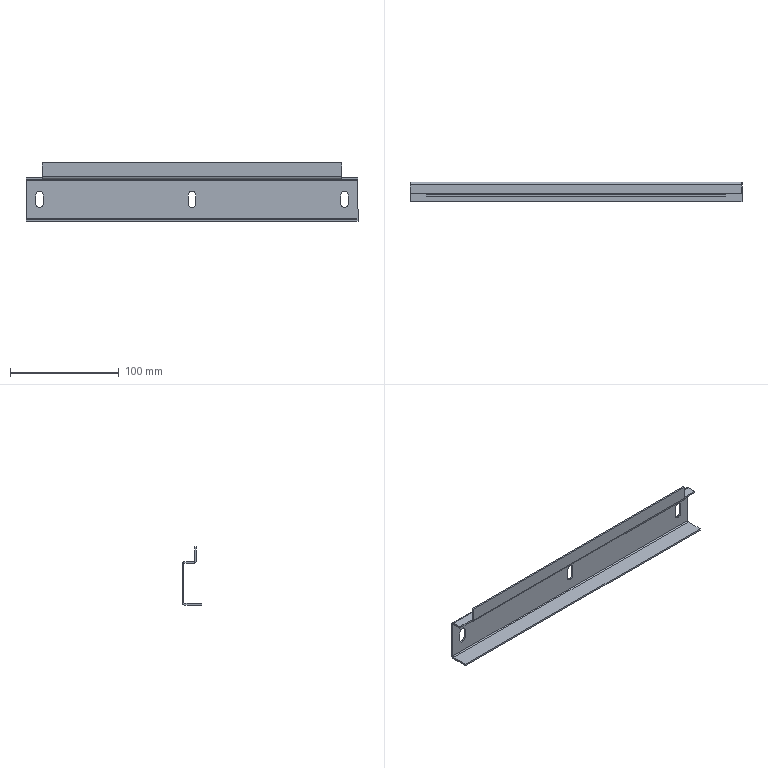Component | SolidWorks | GlassDoorAssembly-1_ShortBentPlate_2-1 | 1 solid | 42 faces | volume 35144 mm3 | plane 30 | cylinder 12 | commonest cylinder face diameters 7 x6 5 x3 2 x3